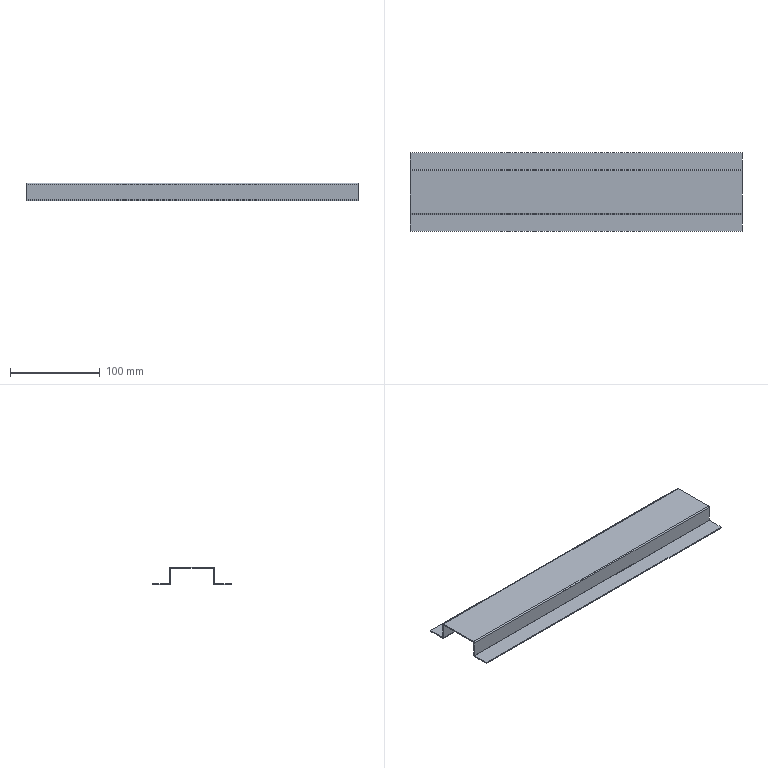Component | SolidWorks | WeldmentDrawing-1_FrontCrossbeam-1 | 1 solid | 38 faces | box 370 x 87.6 x 20 mm | volume 55055 mm3 | plane 30 | cylinder 8 | commonest cylinder face diameters 2.6 x4 0.2 x4
STEP:
#1=CARTESIAN_POINT('',(6.029,-6.77,9.791));
#2=VERTEX_POINT('',#1);
#3=CARTESIAN_POINT('',(6.029,-6.77,9.106));
#4=VERTEX_POINT('',#3);
#5=CARTESIAN_POINT('',(6.029,-6.77,9.795));
#6=DIRECTION('',(0.,-0.,-1.));
#7=VECTOR('',#6,39.37);
#8=LINE('',#5,#7);
#9=EDGE_CURVE('',#2,#4,#8,.T.);
#10=ORIENTED_EDGE('',*,*,#9,.T.);
#11=CARTESIAN_POINT('',(6.029,-6.723,9.106));
#12=VERTEX_POINT('',#11);
#13=CARTESIAN_POINT('',(6.029,-6.77,9.106));
#14=DIRECTION('',(0.,1.,0.));
#15=VECTOR('',#14,39.37);
#16=LINE('',#13,#15);
#17=EDGE_CURVE('',#4,#12,#16,.T.);
#18=ORIENTED_EDGE('',*,*,#17,.T.);
#19=CARTESIAN_POINT('',(6.029,-6.723,9.791));
#20=VERTEX_POINT('',#19);
#21=CARTESIAN_POINT('',(6.029,-6.723,9.843));
#22=DIRECTION('',(0.,-0.,-1.));
#23=VECTOR('',#22,39.37);
#24=LINE('',#21,#23);
#25=EDGE_CURVE('',#20,#12,#24,.T.);
#26=ORIENTED_EDGE('',*,*,#25,.F.);
#27=CARTESIAN_POINT('',(6.029,-6.77,9.791));
#28=DIRECTION('',(0.,-1.,0.));
#29=VECTOR('',#28,39.37);
#30=LINE('',#27,#29);
#31=EDGE_CURVE('',#20,#2,#30,.T.);
#32=ORIENTED_EDGE('',*,*,#31,.T.);
#33=EDGE_LOOP('',(#10,#18,#26,#32));
#34=FACE_OUTER_BOUND('',#33,.T.);
#35=CARTESIAN_POINT('',(6.029,-6.77,9.795));
#36=DIRECTION('',(1.,0.,0.));
#37=DIRECTION('',(0.,0.,-1.));
#38=AXIS2_PLACEMENT_3D('',#35,#36,#37);
#39=PLANE('',#38);
#40=ADVANCED_FACE('',(#34),#39,.T.);
#41=CARTESIAN_POINT('',(-8.538,-6.77,9.106));
#42=VERTEX_POINT('',#41);
#43=CARTESIAN_POINT('',(6.029,-6.77,9.106));
#44=DIRECTION('',(-1.,0.,0.));
#45=VECTOR('',#44,39.37);
#46=LINE('',#43,#45);
#47=EDGE_CURVE('',#4,#42,#46,.T.);
#48=ORIENTED_EDGE('',*,*,#47,.F.);
#49=ORIENTED_EDGE('',*,*,#9,.F.);
#50=CARTESIAN_POINT('',(-8.538,-6.77,9.791));
#51=VERTEX_POINT('',#50);
#52=CARTESIAN_POINT('',(6.029,-6.77,9.791));
#53=DIRECTION('',(1.,-0.,-0.));
#54=VECTOR('',#53,39.37);
#55=LINE('',#52,#54);
#56=EDGE_CURVE('',#51,#2,#55,.T.);
#57=ORIENTED_EDGE('',*,*,#56,.F.);
#58=CARTESIAN_POINT('',(-8.538,-6.77,9.055));
#59=DIRECTION('',(0.,0.,1.));
#60=VECTOR('',#59,39.37);
#61=LINE('',#58,#60);
#62=EDGE_CURVE('',#42,#51,#61,.T.);
#63=ORIENTED_EDGE('',*,*,#62,.F.);
#64=EDGE_LOOP('',(#48,#49,#57,#63));
#65=FACE_OUTER_BOUND('',#64,.T.);
#66=CARTESIAN_POINT('',(-5.572,-6.77,9.843));
#67=DIRECTION('',(0.,1.,-0.));
#68=DIRECTION('',(0.,0.,1.));
#69=AXIS2_PLACEMENT_3D('',#66,#67,#68);
#70=PLANE('',#69);
#71=ADVANCED_FACE('',(#65),#70,.F.);
#72=ORIENTED_EDGE('',*,*,#25,.T.);
#73=CARTESIAN_POINT('',(-8.538,-6.723,9.106));
#74=VERTEX_POINT('',#73);
#75=CARTESIAN_POINT('',(6.029,-6.723,9.106));
#76=DIRECTION('',(-1.,0.,0.));
#77=VECTOR('',#76,39.37);
#78=LINE('',#75,#77);
#79=EDGE_CURVE('',#12,#74,#78,.T.);
#80=ORIENTED_EDGE('',*,*,#79,.T.);
#81=CARTESIAN_POINT('',(-8.538,-6.723,9.791));
#82=VERTEX_POINT('',#81);
#83=CARTESIAN_POINT('',(-8.538,-6.723,9.843));
#84=DIRECTION('',(0.,0.,1.));
#85=VECTOR('',#84,39.37);
#86=LINE('',#83,#85);
#87=EDGE_CURVE('',#74,#82,#86,.T.);
#88=ORIENTED_EDGE('',*,*,#87,.T.);
#89=CARTESIAN_POINT('',(6.029,-6.723,9.791));
#90=DIRECTION('',(-1.,0.,0.));
#91=VECTOR('',#90,39.37);
#92=LINE('',#89,#91);
#93=EDGE_CURVE('',#20,#82,#92,.T.);
#94=ORIENTED_EDGE('',*,*,#93,.F.);
#95=EDGE_LOOP('',(#72,#80,#88,#94));
#96=FACE_OUTER_BOUND('',#95,.T.);
#97=CARTESIAN_POINT('',(-5.572,-6.723,9.843));
#98=DIRECTION('',(0.,1.,-0.));
#99=DIRECTION('',(0.,0.,1.));
#100=AXIS2_PLACEMENT_3D('',#97,#98,#99);
#101=PLANE('',#100);
#102=ADVANCED_FACE('',(#96),#101,.T.);
#103=CARTESIAN_POINT('',(-8.538,-4.801,9.791));
#104=VERTEX_POINT('',#103);
#105=CARTESIAN_POINT('',(-8.538,-4.801,9.106));
#106=VERTEX_POINT('',#105);
#107=CARTESIAN_POINT('',(-8.538,-4.801,9.055));
#108=DIRECTION('',(0.,0.,-1.));
#109=VECTOR('',#108,39.37);
#110=LINE('',#107,#109);
#111=EDGE_CURVE('',#104,#106,#110,.T.);
#112=ORIENTED_EDGE('',*,*,#111,.T.);
#113=CARTESIAN_POINT('',(-8.538,-4.848,9.106));
#114=VERTEX_POINT('',#113);
#115=CARTESIAN_POINT('',(-8.538,-4.801,9.106));
#116=DIRECTION('',(0.,-1.,0.));
#117=VECTOR('',#116,39.37);
#118=LINE('',#115,#117);
#119=EDGE_CURVE('',#106,#114,#118,.T.);
#120=ORIENTED_EDGE('',*,*,#119,.T.);
#121=CARTESIAN_POINT('',(-8.538,-4.848,9.791));
#122=VERTEX_POINT('',#121);
#123=CARTESIAN_POINT('',(-8.538,-4.848,9.843));
#124=DIRECTION('',(0.,0.,-1.));
#125=VECTOR('',#124,39.37);
#126=LINE('',#123,#125);
#127=EDGE_CURVE('',#122,#114,#126,.T.);
#128=ORIENTED_EDGE('',*,*,#127,.F.);
#129=CARTESIAN_POINT('',(-8.538,-4.801,9.791));
#130=DIRECTION('',(0.,1.,0.));
#131=VECTOR('',#130,39.37);
#132=LINE('',#129,#131);
#133=EDGE_CURVE('',#122,#104,#132,.T.);
#134=ORIENTED_EDGE('',*,*,#133,.T.);
#135=EDGE_LOOP('',(#112,#120,#128,#134));
#136=FACE_OUTER_BOUND('',#135,.T.);
#137=CARTESIAN_POINT('',(-8.538,-4.801,9.055));
#138=DIRECTION('',(-1.,0.,0.));
#139=DIRECTION('',(0.,0.,1.));
#140=AXIS2_PLACEMENT_3D('',#137,#138,#139);
#141=PLANE('',#140);
#142=ADVANCED_FACE('',(#136),#141,.T.);
#143=CARTESIAN_POINT('',(6.029,-4.801,9.106));
#144=VERTEX_POINT('',#143);
#145=CARTESIAN_POINT('',(6.029,-4.801,9.791));
#146=VERTEX_POINT('',#145);
#147=CARTESIAN_POINT('',(6.029,-4.801,9.795));
#148=DIRECTION('',(0.,-0.,1.));
#149=VECTOR('',#148,39.37);
#150=LINE('',#147,#149);
#151=EDGE_CURVE('',#144,#146,#150,.T.);
#152=ORIENTED_EDGE('',*,*,#151,.F.);
#153=CARTESIAN_POINT('',(-8.538,-4.801,9.106));
#154=DIRECTION('',(1.,0.,0.));
#155=VECTOR('',#154,39.37);
#156=LINE('',#153,#155);
#157=EDGE_CURVE('',#106,#144,#156,.T.);
#158=ORIENTED_EDGE('',*,*,#157,.F.);
#159=ORIENTED_EDGE('',*,*,#111,.F.);
#160=CARTESIAN_POINT('',(-5.572,-4.801,9.791));
#161=DIRECTION('',(1.,0.,-0.));
#162=VECTOR('',#161,39.37);
#163=LINE('',#160,#162);
#164=EDGE_CURVE('',#104,#146,#163,.T.);
#165=ORIENTED_EDGE('',*,*,#164,.T.);
#166=EDGE_LOOP('',(#152,#158,#159,#165));
#167=FACE_OUTER_BOUND('',#166,.T.);
#168=CARTESIAN_POINT('',(-5.572,-4.801,9.843));
#169=DIRECTION('',(0.,1.,0.));
#170=DIRECTION('',(0.,-0.,1.));
#171=AXIS2_PLACEMENT_3D('',#168,#169,#170);
#172=PLANE('',#171);
#173=ADVANCED_FACE('',(#167),#172,.T.);
#174=CARTESIAN_POINT('',(6.029,-4.848,9.106));
#175=VERTEX_POINT('',#174);
#176=CARTESIAN_POINT('',(-8.538,-4.848,9.106));
#177=DIRECTION('',(1.,0.,0.));
#178=VECTOR('',#177,39.37);
#179=LINE('',#176,#178);
#180=EDGE_CURVE('',#114,#175,#179,.T.);
#181=ORIENTED_EDGE('',*,*,#180,.T.);
#182=CARTESIAN_POINT('',(6.029,-4.848,9.791));
#183=VERTEX_POINT('',#182);
#184=CARTESIAN_POINT('',(6.029,-4.848,9.843));
#185=DIRECTION('',(0.,-0.,1.));
#186=VECTOR('',#185,39.37);
#187=LINE('',#184,#186);
#188=EDGE_CURVE('',#175,#183,#187,.T.);
#189=ORIENTED_EDGE('',*,*,#188,.T.);
#190=CARTESIAN_POINT('',(-8.538,-4.848,9.791));
#191=DIRECTION('',(1.,0.,-0.));
#192=VECTOR('',#191,39.37);
#193=LINE('',#190,#192);
#194=EDGE_CURVE('',#122,#183,#193,.T.);
#195=ORIENTED_EDGE('',*,*,#194,.F.);
#196=ORIENTED_EDGE('',*,*,#127,.T.);
#197=EDGE_LOOP('',(#181,#189,#195,#196));
#198=FACE_OUTER_BOUND('',#197,.T.);
#199=CARTESIAN_POINT('',(-5.572,-4.848,9.843));
#200=DIRECTION('',(0.,1.,0.));
#201=DIRECTION('',(0.,-0.,1.));
#202=AXIS2_PLACEMENT_3D('',#199,#200,#201);
#203=PLANE('',#202);
#204=ADVANCED_FACE('',(#198),#203,.F.);
#205=CARTESIAN_POINT('',(6.029,-6.719,9.795));
#206=VERTEX_POINT('',#205);
#207=CARTESIAN_POINT('',(6.029,-4.852,9.795));
#208=VERTEX_POINT('',#207);
#209=CARTESIAN_POINT('',(6.029,-6.77,9.795));
#210=DIRECTION('',(0.,1.,0.));
#211=VECTOR('',#210,39.37);
#212=LINE('',#209,#211);
#213=EDGE_CURVE('',#206,#208,#212,.T.);
#214=ORIENTED_EDGE('',*,*,#213,.F.);
#215=CARTESIAN_POINT('',(-8.538,-6.719,9.795));
#216=VERTEX_POINT('',#215);
#217=CARTESIAN_POINT('',(-8.538,-6.719,9.795));
#218=DIRECTION('',(1.,0.,0.));
#219=VECTOR('',#218,39.37);
#220=LINE('',#217,#219);
#221=EDGE_CURVE('',#216,#206,#220,.T.);
#222=ORIENTED_EDGE('',*,*,#221,.F.);
#223=CARTESIAN_POINT('',(-8.538,-4.852,9.795));
#224=VERTEX_POINT('',#223);
#225=CARTESIAN_POINT('',(-8.538,-6.77,9.795));
#226=DIRECTION('',(0.,-1.,0.));
#227=VECTOR('',#226,39.37);
#228=LINE('',#225,#227);
#229=EDGE_CURVE('',#224,#216,#228,.T.);
#230=ORIENTED_EDGE('',*,*,#229,.F.);
#231=CARTESIAN_POINT('',(6.029,-4.852,9.795));
#232=DIRECTION('',(-1.,0.,0.));
#233=VECTOR('',#232,39.37);
#234=LINE('',#231,#233);
#235=EDGE_CURVE('',#208,#224,#234,.T.);
#236=ORIENTED_EDGE('',*,*,#235,.F.);
#237=EDGE_LOOP('',(#214,#222,#230,#236));
#238=FACE_OUTER_BOUND('',#237,.T.);
#239=CARTESIAN_POINT('',(-5.572,-6.661,9.795));
#240=DIRECTION('',(0.,0.,-1.));
#241=DIRECTION('',(-1.,0.,0.));
#242=AXIS2_PLACEMENT_3D('',#239,#240,#241);
#243=PLANE('',#242);
#244=ADVANCED_FACE('',(#238),#243,.T.);
#245=CARTESIAN_POINT('',(-8.538,-6.719,9.843));
#246=VERTEX_POINT('',#245);
#247=CARTESIAN_POINT('',(6.029,-6.719,9.843));
#248=VERTEX_POINT('',#247);
#249=CARTESIAN_POINT('',(-8.538,-6.719,9.843));
#250=DIRECTION('',(1.,0.,0.));
#251=VECTOR('',#250,39.37);
#252=LINE('',#249,#251);
#253=EDGE_CURVE('',#246,#248,#252,.T.);
#254=ORIENTED_EDGE('',*,*,#253,.T.);
#255=CARTESIAN_POINT('',(6.029,-4.852,9.843));
#256=VERTEX_POINT('',#255);
#257=CARTESIAN_POINT('',(6.029,-6.77,9.843));
#258=DIRECTION('',(0.,1.,0.));
#259=VECTOR('',#258,39.37);
#260=LINE('',#257,#259);
#261=EDGE_CURVE('',#248,#256,#260,.T.);
#262=ORIENTED_EDGE('',*,*,#261,.T.);
#263=CARTESIAN_POINT('',(-8.538,-4.852,9.843));
#264=VERTEX_POINT('',#263);
#265=CARTESIAN_POINT('',(6.029,-4.852,9.843));
#266=DIRECTION('',(-1.,0.,0.));
#267=VECTOR('',#266,39.37);
#268=LINE('',#265,#267);
#269=EDGE_CURVE('',#256,#264,#268,.T.);
#270=ORIENTED_EDGE('',*,*,#269,.T.);
#271=CARTESIAN_POINT('',(-8.538,-6.77,9.843));
#272=DIRECTION('',(0.,-1.,0.));
#273=VECTOR('',#272,39.37);
#274=LINE('',#271,#273);
#275=EDGE_CURVE('',#264,#246,#274,.T.);
#276=ORIENTED_EDGE('',*,*,#275,.T.);
#277=EDGE_LOOP('',(#254,#262,#270,#276));
#278=FACE_OUTER_BOUND('',#277,.T.);
#279=CARTESIAN_POINT('',(-5.572,-6.661,9.843));
#280=DIRECTION('',(0.,0.,-1.));
#281=DIRECTION('',(-1.,0.,0.));
#282=AXIS2_PLACEMENT_3D('',#279,#280,#281);
#283=PLANE('',#282);
#284=ADVANCED_FACE('',(#278),#283,.F.);
#285=ORIENTED_EDGE('',*,*,#229,.T.);
#286=CARTESIAN_POINT('',(-8.538,-6.719,9.795));
#287=DIRECTION('',(0.,0.,1.));
#288=VECTOR('',#287,39.37);
#289=LINE('',#286,#288);
#290=EDGE_CURVE('',#216,#246,#289,.T.);
#291=ORIENTED_EDGE('',*,*,#290,.T.);
#292=ORIENTED_EDGE('',*,*,#275,.F.);
#293=CARTESIAN_POINT('',(-8.538,-4.852,9.795));
#294=DIRECTION('',(0.,0.,1.));
#295=VECTOR('',#294,39.37);
#296=LINE('',#293,#295);
#297=EDGE_CURVE('',#224,#264,#296,.T.);
#298=ORIENTED_EDGE('',*,*,#297,.F.);
#299=EDGE_LOOP('',(#285,#291,#292,#298));
#300=FACE_OUTER_BOUND('',#299,.T.);
#301=CARTESIAN_POINT('',(-8.538,-6.77,9.795));
#302=DIRECTION('',(-1.,0.,0.));
#303=DIRECTION('',(0.,0.,1.));
#304=AXIS2_PLACEMENT_3D('',#301,#302,#303);
#305=PLANE('',#304);
#306=ADVANCED_FACE('',(#300),#305,.T.);
#307=CARTESIAN_POINT('',(6.029,-6.719,9.795));
#308=DIRECTION('',(0.,0.,1.));
#309=VECTOR('',#308,39.37);
#310=LINE('',#307,#309);
#311=EDGE_CURVE('',#206,#248,#310,.T.);
#312=ORIENTED_EDGE('',*,*,#311,.F.);
#313=ORIENTED_EDGE('',*,*,#213,.T.);
#314=CARTESIAN_POINT('',(6.029,-4.852,9.795));
#315=DIRECTION('',(0.,0.,1.));
#316=VECTOR('',#315,39.37);
#317=LINE('',#314,#316);
#318=EDGE_CURVE('',#208,#256,#317,.T.);
#319=ORIENTED_EDGE('',*,*,#318,.T.);
#320=ORIENTED_EDGE('',*,*,#261,.F.);
#321=EDGE_LOOP('',(#312,#313,#319,#320));
#322=FACE_OUTER_BOUND('',#321,.T.);
#323=CARTESIAN_POINT('',(6.029,-6.77,9.795));
#324=DIRECTION('',(1.,0.,0.));
#325=DIRECTION('',(0.,0.,-1.));
#326=AXIS2_PLACEMENT_3D('',#323,#324,#325);
#327=PLANE('',#326);
#328=ADVANCED_FACE('',(#322),#327,.T.);
#329=ORIENTED_EDGE('',*,*,#133,.F.);
#330=CARTESIAN_POINT('',(-8.538,-4.852,9.791));
#331=DIRECTION('',(-1.,0.,0.));
#332=DIRECTION('',(0.,0.,-1.));
#333=AXIS2_PLACEMENT_3D('',#330,#331,#332);
#334=CIRCLE('',#333,0.003937);
#335=EDGE_CURVE('',#224,#122,#334,.T.);
#336=ORIENTED_EDGE('',*,*,#335,.F.);
#337=ORIENTED_EDGE('',*,*,#297,.T.);
#338=CARTESIAN_POINT('',(-8.538,-4.852,9.791));
#339=DIRECTION('',(-1.,0.,0.));
#340=DIRECTION('',(0.,0.,-1.));
#341=AXIS2_PLACEMENT_3D('',#338,#339,#340);
#342=CIRCLE('',#341,0.05118);
#343=EDGE_CURVE('',#264,#104,#342,.T.);
#344=ORIENTED_EDGE('',*,*,#343,.T.);
#345=EDGE_LOOP('',(#329,#336,#337,#344));
#346=FACE_OUTER_BOUND('',#345,.T.);
#347=CARTESIAN_POINT('',(-8.538,-4.852,9.791));
#348=DIRECTION('',(-1.,0.,0.));
#349=DIRECTION('',(0.,0.,1.));
#350=AXIS2_PLACEMENT_3D('',#347,#348,#349);
#351=PLANE('',#350);
#352=ADVANCED_FACE('',(#346),#351,.T.);
#353=CARTESIAN_POINT('',(6.029,-4.852,9.791));
#354=DIRECTION('',(1.,0.,0.));
#355=DIRECTION('',(0.,0.,-1.));
#356=AXIS2_PLACEMENT_3D('',#353,#354,#355);
#357=CIRCLE('',#356,0.003937);
#358=EDGE_CURVE('',#183,#208,#357,.T.);
#359=ORIENTED_EDGE('',*,*,#358,.F.);
#360=CARTESIAN_POINT('',(6.029,-4.848,9.791));
#361=DIRECTION('',(0.,1.,0.));
#362=VECTOR('',#361,39.37);
#363=LINE('',#360,#362);
#364=EDGE_CURVE('',#183,#146,#363,.T.);
#365=ORIENTED_EDGE('',*,*,#364,.T.);
#366=CARTESIAN_POINT('',(6.029,-4.852,9.791));
#367=DIRECTION('',(1.,0.,0.));
#368=DIRECTION('',(0.,0.,-1.));
#369=AXIS2_PLACEMENT_3D('',#366,#367,#368);
#370=CIRCLE('',#369,0.05118);
#371=EDGE_CURVE('',#146,#256,#370,.T.);
#372=ORIENTED_EDGE('',*,*,#371,.T.);
#373=ORIENTED_EDGE('',*,*,#318,.F.);
#374=EDGE_LOOP('',(#359,#365,#372,#373));
#375=FACE_OUTER_BOUND('',#374,.T.);
#376=CARTESIAN_POINT('',(6.029,-4.852,9.791));
#377=DIRECTION('',(-1.,0.,0.));
#378=DIRECTION('',(0.,0.,1.));
#379=AXIS2_PLACEMENT_3D('',#376,#377,#378);
#380=PLANE('',#379);
#381=ADVANCED_FACE('',(#375),#380,.F.);
#382=ORIENTED_EDGE('',*,*,#269,.F.);
#383=ORIENTED_EDGE('',*,*,#371,.F.);
#384=ORIENTED_EDGE('',*,*,#164,.F.);
#385=ORIENTED_EDGE('',*,*,#343,.F.);
#386=EDGE_LOOP('',(#382,#383,#384,#385));
#387=FACE_OUTER_BOUND('',#386,.T.);
#388=CARTESIAN_POINT('',(6.029,-4.852,9.791));
#389=DIRECTION('',(1.,0.,0.));
#390=DIRECTION('',(0.,1.,0.));
#391=AXIS2_PLACEMENT_3D('',#388,#389,#390);
#392=CYLINDRICAL_SURFACE('',#391,0.05118);
#393=ADVANCED_FACE('',(#387),#392,.T.);
#394=ORIENTED_EDGE('',*,*,#235,.T.);
#395=ORIENTED_EDGE('',*,*,#335,.T.);
#396=ORIENTED_EDGE('',*,*,#194,.T.);
#397=ORIENTED_EDGE('',*,*,#358,.T.);
#398=EDGE_LOOP('',(#394,#395,#396,#397));
#399=FACE_OUTER_BOUND('',#398,.T.);
#400=CARTESIAN_POINT('',(6.029,-4.852,9.791));
#401=DIRECTION('',(1.,0.,0.));
#402=DIRECTION('',(0.,1.,0.));
#403=AXIS2_PLACEMENT_3D('',#400,#401,#402);
#404=CYLINDRICAL_SURFACE('',#403,0.003937);
#405=ADVANCED_FACE('',(#399),#404,.F.);
#406=CARTESIAN_POINT('',(6.029,-4.801,9.106));
#407=DIRECTION('',(0.,-1.,0.));
#408=VECTOR('',#407,39.37);
#409=LINE('',#406,#408);
#410=EDGE_CURVE('',#144,#175,#409,.T.);
#411=ORIENTED_EDGE('',*,*,#410,.F.);
#412=ORIENTED_EDGE('',*,*,#151,.T.);
#413=ORIENTED_EDGE('',*,*,#364,.F.);
#414=ORIENTED_EDGE('',*,*,#188,.F.);
#415=EDGE_LOOP('',(#411,#412,#413,#414));
#416=FACE_OUTER_BOUND('',#415,.T.);
#417=CARTESIAN_POINT('',(6.029,-4.801,9.795));
#418=DIRECTION('',(1.,0.,0.));
#419=DIRECTION('',(0.,0.,-1.));
#420=AXIS2_PLACEMENT_3D('',#417,#418,#419);
#421=PLANE('',#420);
#422=ADVANCED_FACE('',(#416),#421,.T.);
#423=ORIENTED_EDGE('',*,*,#31,.F.);
#424=CARTESIAN_POINT('',(6.029,-6.719,9.791));
#425=DIRECTION('',(1.,0.,0.));
#426=DIRECTION('',(0.,0.,1.));
#427=AXIS2_PLACEMENT_3D('',#424,#425,#426);
#428=CIRCLE('',#427,0.003937);
#429=EDGE_CURVE('',#206,#20,#428,.T.);
#430=ORIENTED_EDGE('',*,*,#429,.F.);
#431=ORIENTED_EDGE('',*,*,#311,.T.);
#432=CARTESIAN_POINT('',(6.029,-6.719,9.791));
#433=DIRECTION('',(1.,0.,0.));
#434=DIRECTION('',(0.,0.,1.));
#435=AXIS2_PLACEMENT_3D('',#432,#433,#434);
#436=CIRCLE('',#435,0.05118);
#437=EDGE_CURVE('',#248,#2,#436,.T.);
#438=ORIENTED_EDGE('',*,*,#437,.T.);
#439=EDGE_LOOP('',(#423,#430,#431,#438));
#440=FACE_OUTER_BOUND('',#439,.T.);
#441=CARTESIAN_POINT('',(6.029,-6.719,9.791));
#442=DIRECTION('',(1.,0.,0.));
#443=DIRECTION('',(0.,0.,-1.));
#444=AXIS2_PLACEMENT_3D('',#441,#442,#443);
#445=PLANE('',#444);
#446=ADVANCED_FACE('',(#440),#445,.T.);
#447=CARTESIAN_POINT('',(-8.538,-6.719,9.791));
#448=DIRECTION('',(-1.,0.,0.));
#449=DIRECTION('',(0.,0.,1.));
#450=AXIS2_PLACEMENT_3D('',#447,#448,#449);
#451=CIRCLE('',#450,0.003937);
#452=EDGE_CURVE('',#82,#216,#451,.T.);
#453=ORIENTED_EDGE('',*,*,#452,.F.);
#454=CARTESIAN_POINT('',(-8.538,-6.723,9.791));
#455=DIRECTION('',(0.,-1.,0.));
#456=VECTOR('',#455,39.37);
#457=LINE('',#454,#456);
#458=EDGE_CURVE('',#82,#51,#457,.T.);
#459=ORIENTED_EDGE('',*,*,#458,.T.);
#460=CARTESIAN_POINT('',(-8.538,-6.719,9.791));
#461=DIRECTION('',(-1.,0.,0.));
#462=DIRECTION('',(0.,0.,1.));
#463=AXIS2_PLACEMENT_3D('',#460,#461,#462);
#464=CIRCLE('',#463,0.05118);
#465=EDGE_CURVE('',#51,#246,#464,.T.);
#466=ORIENTED_EDGE('',*,*,#465,.T.);
#467=ORIENTED_EDGE('',*,*,#290,.F.);
#468=EDGE_LOOP('',(#453,#459,#466,#467));
#469=FACE_OUTER_BOUND('',#468,.T.);
#470=CARTESIAN_POINT('',(-8.538,-6.719,9.791));
#471=DIRECTION('',(1.,0.,0.));
#472=DIRECTION('',(0.,0.,-1.));
#473=AXIS2_PLACEMENT_3D('',#470,#471,#472);
#474=PLANE('',#473);
#475=ADVANCED_FACE('',(#469),#474,.F.);
#476=ORIENTED_EDGE('',*,*,#253,.F.);
#477=ORIENTED_EDGE('',*,*,#465,.F.);
#478=ORIENTED_EDGE('',*,*,#56,.T.);
#479=ORIENTED_EDGE('',*,*,#437,.F.);
#480=EDGE_LOOP('',(#476,#477,#478,#479));
#481=FACE_OUTER_BOUND('',#480,.T.);
#482=CARTESIAN_POINT('',(-8.538,-6.719,9.791));
#483=DIRECTION('',(-1.,0.,0.));
#484=DIRECTION('',(0.,-1.,0.));
#485=AXIS2_PLACEMENT_3D('',#482,#483,#484);
#486=CYLINDRICAL_SURFACE('',#485,0.05118);
#487=ADVANCED_FACE('',(#481),#486,.T.);
#488=ORIENTED_EDGE('',*,*,#221,.T.);
#489=ORIENTED_EDGE('',*,*,#429,.T.);
#490=ORIENTED_EDGE('',*,*,#93,.T.);
#491=ORIENTED_EDGE('',*,*,#452,.T.);
#492=EDGE_LOOP('',(#488,#489,#490,#491));
#493=FACE_OUTER_BOUND('',#492,.T.);
#494=CARTESIAN_POINT('',(-8.538,-6.719,9.791));
#495=DIRECTION('',(-1.,0.,0.));
#496=DIRECTION('',(0.,-1.,0.));
#497=AXIS2_PLACEMENT_3D('',#494,#495,#496);
#498=CYLINDRICAL_SURFACE('',#497,0.003937);
#499=ADVANCED_FACE('',(#493),#498,.F.);
#500=CARTESIAN_POINT('',(-8.538,-6.77,9.106));
#501=DIRECTION('',(0.,1.,0.));
#502=VECTOR('',#501,39.37);
#503=LINE('',#500,#502);
#504=EDGE_CURVE('',#42,#74,#503,.T.);
#505=ORIENTED_EDGE('',*,*,#504,.F.);
#506=ORIENTED_EDGE('',*,*,#62,.T.);
#507=ORIENTED_EDGE('',*,*,#458,.F.);
#508=ORIENTED_EDGE('',*,*,#87,.F.);
#509=EDGE_LOOP('',(#505,#506,#507,#508));
#510=FACE_OUTER_BOUND('',#509,.T.);
#511=CARTESIAN_POINT('',(-8.538,-6.77,9.055));
#512=DIRECTION('',(-1.,0.,0.));
#513=DIRECTION('',(0.,0.,1.));
#514=AXIS2_PLACEMENT_3D('',#511,#512,#513);
#515=PLANE('',#514);
#516=ADVANCED_FACE('',(#510),#515,.T.);
#517=CARTESIAN_POINT('',(6.029,-4.797,9.102));
#518=VERTEX_POINT('',#517);
#519=CARTESIAN_POINT('',(6.029,-4.797,9.055));
#520=VERTEX_POINT('',#519);
#521=CARTESIAN_POINT('',(6.029,-4.797,9.055));
#522=DIRECTION('',(0.,0.,-1.));
#523=VECTOR('',#522,39.37);
#524=LINE('',#521,#523);
#525=EDGE_CURVE('',#518,#520,#524,.T.);
#526=ORIENTED_EDGE('',*,*,#525,.F.);
#527=CARTESIAN_POINT('',(6.029,-4.797,9.106));
#528=DIRECTION('',(1.,0.,0.));
#529=DIRECTION('',(0.,0.,1.));
#530=AXIS2_PLACEMENT_3D('',#527,#528,#529);
#531=CIRCLE('',#530,0.003937);
#532=EDGE_CURVE('',#144,#518,#531,.T.);
#533=ORIENTED_EDGE('',*,*,#532,.F.);
#534=ORIENTED_EDGE('',*,*,#410,.T.);
#535=CARTESIAN_POINT('',(6.029,-4.797,9.106));
#536=DIRECTION('',(1.,0.,0.));
#537=DIRECTION('',(0.,0.,1.));
#538=AXIS2_PLACEMENT_3D('',#535,#536,#537);
#539=CIRCLE('',#538,0.05118);
#540=EDGE_CURVE('',#175,#520,#539,.T.);
#541=ORIENTED_EDGE('',*,*,#540,.T.);
#542=EDGE_LOOP('',(#526,#533,#534,#541));
#543=FACE_OUTER_BOUND('',#542,.T.);
#544=CARTESIAN_POINT('',(6.029,-4.797,9.106));
#545=DIRECTION('',(1.,0.,0.));
#546=DIRECTION('',(0.,0.,-1.));
#547=AXIS2_PLACEMENT_3D('',#544,#545,#546);
#548=PLANE('',#547);
#549=ADVANCED_FACE('',(#543),#548,.T.);
#550=CARTESIAN_POINT('',(-8.538,-4.797,9.102));
#551=VERTEX_POINT('',#550);
#552=CARTESIAN_POINT('',(-8.538,-4.797,9.106));
#553=DIRECTION('',(-1.,0.,0.));
#554=DIRECTION('',(0.,0.,1.));
#555=AXIS2_PLACEMENT_3D('',#552,#553,#554);
#556=CIRCLE('',#555,0.003937);
#557=EDGE_CURVE('',#551,#106,#556,.T.);
#558=ORIENTED_EDGE('',*,*,#557,.F.);
#559=CARTESIAN_POINT('',(-8.538,-4.797,9.055));
#560=VERTEX_POINT('',#559);
#561=CARTESIAN_POINT('',(-8.538,-4.797,9.102));
#562=DIRECTION('',(0.,0.,-1.));
#563=VECTOR('',#562,39.37);
#564=LINE('',#561,#563);
#565=EDGE_CURVE('',#551,#560,#564,.T.);
#566=ORIENTED_EDGE('',*,*,#565,.T.);
#567=CARTESIAN_POINT('',(-8.538,-4.797,9.106));
#568=DIRECTION('',(-1.,0.,0.));
#569=DIRECTION('',(0.,0.,1.));
#570=AXIS2_PLACEMENT_3D('',#567,#568,#569);
#571=CIRCLE('',#570,0.05118);
#572=EDGE_CURVE('',#560,#114,#571,.T.);
#573=ORIENTED_EDGE('',*,*,#572,.T.);
#574=ORIENTED_EDGE('',*,*,#119,.F.);
#575=EDGE_LOOP('',(#558,#566,#573,#574));
#576=FACE_OUTER_BOUND('',#575,.T.);
#577=CARTESIAN_POINT('',(-8.538,-4.797,9.106));
#578=DIRECTION('',(1.,0.,0.));
#579=DIRECTION('',(0.,0.,-1.));
#580=AXIS2_PLACEMENT_3D('',#577,#578,#579);
#581=PLANE('',#580);
#582=ADVANCED_FACE('',(#576),#581,.F.);
#583=ORIENTED_EDGE('',*,*,#180,.F.);
#584=ORIENTED_EDGE('',*,*,#572,.F.);
#585=CARTESIAN_POINT('',(6.029,-4.797,9.055));
#586=DIRECTION('',(1.,0.,0.));
#587=VECTOR('',#586,39.37);
#588=LINE('',#585,#587);
#589=EDGE_CURVE('',#560,#520,#588,.T.);
#590=ORIENTED_EDGE('',*,*,#589,.T.);
#591=ORIENTED_EDGE('',*,*,#540,.F.);
#592=EDGE_LOOP('',(#583,#584,#590,#591));
#593=FACE_OUTER_BOUND('',#592,.T.);
#594=CARTESIAN_POINT('',(-8.538,-4.797,9.106));
#595=DIRECTION('',(-1.,0.,0.));
#596=DIRECTION('',(0.,0.,-1.));
#597=AXIS2_PLACEMENT_3D('',#594,#595,#596);
#598=CYLINDRICAL_SURFACE('',#597,0.05118);
#599=ADVANCED_FACE('',(#593),#598,.T.);
#600=ORIENTED_EDGE('',*,*,#157,.T.);
#601=ORIENTED_EDGE('',*,*,#532,.T.);
#602=CARTESIAN_POINT('',(6.029,-4.797,9.102));
#603=DIRECTION('',(-1.,0.,0.));
#604=VECTOR('',#603,39.37);
#605=LINE('',#602,#604);
#606=EDGE_CURVE('',#518,#551,#605,.T.);
#607=ORIENTED_EDGE('',*,*,#606,.T.);
#608=ORIENTED_EDGE('',*,*,#557,.T.);
#609=EDGE_LOOP('',(#600,#601,#607,#608));
#610=FACE_OUTER_BOUND('',#609,.T.);
#611=CARTESIAN_POINT('',(-8.538,-4.797,9.106));
#612=DIRECTION('',(-1.,0.,0.));
#613=DIRECTION('',(0.,0.,-1.));
#614=AXIS2_PLACEMENT_3D('',#611,#612,#613);
#615=CYLINDRICAL_SURFACE('',#614,0.003937);
#616=ADVANCED_FACE('',(#610),#615,.F.);
#617=ORIENTED_EDGE('',*,*,#565,.F.);
#618=CARTESIAN_POINT('',(-8.538,-4.061,9.102));
#619=VERTEX_POINT('',#618);
#620=CARTESIAN_POINT('',(-8.538,-4.061,9.102));
#621=DIRECTION('',(0.,1.,-0.));
#622=VECTOR('',#621,39.37);
#623=LINE('',#620,#622);
#624=EDGE_CURVE('',#551,#619,#623,.T.);
#625=ORIENTED_EDGE('',*,*,#624,.T.);
#626=CARTESIAN_POINT('',(-8.538,-4.061,9.055));
#627=VERTEX_POINT('',#626);
#628=CARTESIAN_POINT('',(-8.538,-4.061,9.055));
#629=DIRECTION('',(0.,0.,1.));
#630=VECTOR('',#629,39.37);
#631=LINE('',#628,#630);
#632=EDGE_CURVE('',#627,#619,#631,.T.);
#633=ORIENTED_EDGE('',*,*,#632,.F.);
#634=CARTESIAN_POINT('',(-8.538,-6.661,9.055));
#635=DIRECTION('',(0.,1.,-0.));
#636=VECTOR('',#635,39.37);
#637=LINE('',#634,#636);
#638=EDGE_CURVE('',#560,#627,#637,.T.);
#639=ORIENTED_EDGE('',*,*,#638,.F.);
#640=EDGE_LOOP('',(#617,#625,#633,#639));
#641=FACE_OUTER_BOUND('',#640,.T.);
#642=CARTESIAN_POINT('',(-8.538,-4.061,9.055));
#643=DIRECTION('',(1.,0.,0.));
#644=DIRECTION('',(0.,0.,-1.));
#645=AXIS2_PLACEMENT_3D('',#642,#643,#644);
#646=PLANE('',#645);
#647=ADVANCED_FACE('',(#641),#646,.F.);
#648=ORIENTED_EDGE('',*,*,#525,.T.);
#649=CARTESIAN_POINT('',(6.029,-4.061,9.055));
#650=VERTEX_POINT('',#649);
#651=CARTESIAN_POINT('',(6.029,-6.661,9.055));
#652=DIRECTION('',(0.,-1.,0.));
#653=VECTOR('',#652,39.37);
#654=LINE('',#651,#653);
#655=EDGE_CURVE('',#650,#520,#654,.T.);
#656=ORIENTED_EDGE('',*,*,#655,.F.);
#657=CARTESIAN_POINT('',(6.029,-4.061,9.102));
#658=VERTEX_POINT('',#657);
#659=CARTESIAN_POINT('',(6.029,-4.061,9.055));
#660=DIRECTION('',(0.,0.,1.));
#661=VECTOR('',#660,39.37);
#662=LINE('',#659,#661);
#663=EDGE_CURVE('',#650,#658,#662,.T.);
#664=ORIENTED_EDGE('',*,*,#663,.T.);
#665=CARTESIAN_POINT('',(6.029,-4.801,9.102));
#666=DIRECTION('',(0.,-1.,0.));
#667=VECTOR('',#666,39.37);
#668=LINE('',#665,#667);
#669=EDGE_CURVE('',#658,#518,#668,.T.);
#670=ORIENTED_EDGE('',*,*,#669,.T.);
#671=EDGE_LOOP('',(#648,#656,#664,#670));
#672=FACE_OUTER_BOUND('',#671,.T.);
#673=CARTESIAN_POINT('',(6.029,-4.801,9.055));
#674=DIRECTION('',(-1.,0.,0.));
#675=DIRECTION('',(0.,0.,1.));
#676=AXIS2_PLACEMENT_3D('',#673,#674,#675);
#677=PLANE('',#676);
#678=ADVANCED_FACE('',(#672),#677,.F.);
#679=ORIENTED_EDGE('',*,*,#589,.F.);
#680=ORIENTED_EDGE('',*,*,#638,.T.);
#681=CARTESIAN_POINT('',(-5.572,-4.061,9.055));
#682=DIRECTION('',(1.,0.,0.));
#683=VECTOR('',#682,39.37);
#684=LINE('',#681,#683);
#685=EDGE_CURVE('',#627,#650,#684,.T.);
#686=ORIENTED_EDGE('',*,*,#685,.T.);
#687=ORIENTED_EDGE('',*,*,#655,.T.);
#688=EDGE_LOOP('',(#679,#680,#686,#687));
#689=FACE_OUTER_BOUND('',#688,.T.);
#690=CARTESIAN_POINT('',(-5.572,-6.661,9.055));
#691=DIRECTION('',(0.,0.,1.));
#692=DIRECTION('',(0.,-1.,0.));
#693=AXIS2_PLACEMENT_3D('',#690,#691,#692);
#694=PLANE('',#693);
#695=ADVANCED_FACE('',(#689),#694,.F.);
#696=ORIENTED_EDGE('',*,*,#624,.F.);
#697=ORIENTED_EDGE('',*,*,#606,.F.);
#698=ORIENTED_EDGE('',*,*,#669,.F.);
#699=CARTESIAN_POINT('',(6.029,-4.061,9.102));
#700=DIRECTION('',(1.,0.,0.));
#701=VECTOR('',#700,39.37);
#702=LINE('',#699,#701);
#703=EDGE_CURVE('',#619,#658,#702,.T.);
#704=ORIENTED_EDGE('',*,*,#703,.F.);
#705=EDGE_LOOP('',(#696,#697,#698,#704));
#706=FACE_OUTER_BOUND('',#705,.T.);
#707=CARTESIAN_POINT('',(-5.572,-6.661,9.102));
#708=DIRECTION('',(0.,0.,1.));
#709=DIRECTION('',(0.,-1.,0.));
#710=AXIS2_PLACEMENT_3D('',#707,#708,#709);
#711=PLANE('',#710);
#712=ADVANCED_FACE('',(#706),#711,.T.);
#713=ORIENTED_EDGE('',*,*,#703,.T.);
#714=ORIENTED_EDGE('',*,*,#663,.F.);
#715=ORIENTED_EDGE('',*,*,#685,.F.);
#716=ORIENTED_EDGE('',*,*,#632,.T.);
#717=EDGE_LOOP('',(#713,#714,#715,#716));
#718=FACE_OUTER_BOUND('',#717,.T.);
#719=CARTESIAN_POINT('',(6.029,-4.061,9.055));
#720=DIRECTION('',(0.,-1.,0.));
#721=DIRECTION('',(0.,-0.,-1.));
#722=AXIS2_PLACEMENT_3D('',#719,#720,#721);
#723=PLANE('',#722);
#724=ADVANCED_FACE('',(#718),#723,.F.);
#725=CARTESIAN_POINT('',(-8.538,-6.774,9.102));
#726=VERTEX_POINT('',#725);
#727=CARTESIAN_POINT('',(-8.538,-6.774,9.055));
#728=VERTEX_POINT('',#727);
#729=CARTESIAN_POINT('',(-8.538,-6.774,9.055));
#730=DIRECTION('',(0.,0.,-1.));
#731=VECTOR('',#730,39.37);
#732=LINE('',#729,#731);
#733=EDGE_CURVE('',#726,#728,#732,.T.);
#734=ORIENTED_EDGE('',*,*,#733,.F.);
#735=CARTESIAN_POINT('',(-8.538,-6.774,9.106));
#736=DIRECTION('',(-1.,0.,0.));
#737=DIRECTION('',(0.,0.,-1.));
#738=AXIS2_PLACEMENT_3D('',#735,#736,#737);
#739=CIRCLE('',#738,0.003937);
#740=EDGE_CURVE('',#42,#726,#739,.T.);
#741=ORIENTED_EDGE('',*,*,#740,.F.);
#742=ORIENTED_EDGE('',*,*,#504,.T.);
#743=CARTESIAN_POINT('',(-8.538,-6.774,9.106));
#744=DIRECTION('',(-1.,0.,0.));
#745=DIRECTION('',(0.,0.,-1.));
#746=AXIS2_PLACEMENT_3D('',#743,#744,#745);
#747=CIRCLE('',#746,0.05118);
#748=EDGE_CURVE('',#74,#728,#747,.T.);
#749=ORIENTED_EDGE('',*,*,#748,.T.);
#750=EDGE_LOOP('',(#734,#741,#742,#749));
#751=FACE_OUTER_BOUND('',#750,.T.);
#752=CARTESIAN_POINT('',(-8.538,-6.774,9.106));
#753=DIRECTION('',(-1.,0.,0.));
#754=DIRECTION('',(0.,0.,1.));
#755=AXIS2_PLACEMENT_3D('',#752,#753,#754);
#756=PLANE('',#755);
#757=ADVANCED_FACE('',(#751),#756,.T.);
#758=CARTESIAN_POINT('',(6.029,-6.774,9.102));
#759=VERTEX_POINT('',#758);
#760=CARTESIAN_POINT('',(6.029,-6.774,9.106));
#761=DIRECTION('',(1.,0.,0.));
#762=DIRECTION('',(0.,0.,-1.));
#763=AXIS2_PLACEMENT_3D('',#760,#761,#762);
#764=CIRCLE('',#763,0.003937);
#765=EDGE_CURVE('',#759,#4,#764,.T.);
#766=ORIENTED_EDGE('',*,*,#765,.F.);
#767=CARTESIAN_POINT('',(6.029,-6.774,9.055));
#768=VERTEX_POINT('',#767);
#769=CARTESIAN_POINT('',(6.029,-6.774,9.102));
#770=DIRECTION('',(0.,0.,-1.));
#771=VECTOR('',#770,39.37);
#772=LINE('',#769,#771);
#773=EDGE_CURVE('',#759,#768,#772,.T.);
#774=ORIENTED_EDGE('',*,*,#773,.T.);
#775=CARTESIAN_POINT('',(6.029,-6.774,9.106));
#776=DIRECTION('',(1.,0.,0.));
#777=DIRECTION('',(0.,0.,-1.));
#778=AXIS2_PLACEMENT_3D('',#775,#776,#777);
#779=CIRCLE('',#778,0.05118);
#780=EDGE_CURVE('',#768,#12,#779,.T.);
#781=ORIENTED_EDGE('',*,*,#780,.T.);
#782=ORIENTED_EDGE('',*,*,#17,.F.);
#783=EDGE_LOOP('',(#766,#774,#781,#782));
#784=FACE_OUTER_BOUND('',#783,.T.);
#785=CARTESIAN_POINT('',(6.029,-6.774,9.106));
#786=DIRECTION('',(-1.,0.,0.));
#787=DIRECTION('',(0.,0.,1.));
#788=AXIS2_PLACEMENT_3D('',#785,#786,#787);
#789=PLANE('',#788);
#790=ADVANCED_FACE('',(#784),#789,.F.);
#791=ORIENTED_EDGE('',*,*,#79,.F.);
#792=ORIENTED_EDGE('',*,*,#780,.F.);
#793=CARTESIAN_POINT('',(-8.538,-6.774,9.055));
#794=DIRECTION('',(-1.,-0.,0.));
#795=VECTOR('',#794,39.37);
#796=LINE('',#793,#795);
#797=EDGE_CURVE('',#768,#728,#796,.T.);
#798=ORIENTED_EDGE('',*,*,#797,.T.);
#799=ORIENTED_EDGE('',*,*,#748,.F.);
#800=EDGE_LOOP('',(#791,#792,#798,#799));
#801=FACE_OUTER_BOUND('',#800,.T.);
#802=CARTESIAN_POINT('',(6.029,-6.774,9.106));
#803=DIRECTION('',(1.,0.,0.));
#804=DIRECTION('',(0.,0.,-1.));
#805=AXIS2_PLACEMENT_3D('',#802,#803,#804);
#806=CYLINDRICAL_SURFACE('',#805,0.05118);
#807=ADVANCED_FACE('',(#801),#806,.T.);
#808=ORIENTED_EDGE('',*,*,#47,.T.);
#809=ORIENTED_EDGE('',*,*,#740,.T.);
#810=CARTESIAN_POINT('',(-8.538,-6.774,9.102));
#811=DIRECTION('',(1.,0.,0.));
#812=VECTOR('',#811,39.37);
#813=LINE('',#810,#812);
#814=EDGE_CURVE('',#726,#759,#813,.T.);
#815=ORIENTED_EDGE('',*,*,#814,.T.);
#816=ORIENTED_EDGE('',*,*,#765,.T.);
#817=EDGE_LOOP('',(#808,#809,#815,#816));
#818=FACE_OUTER_BOUND('',#817,.T.);
#819=CARTESIAN_POINT('',(6.029,-6.774,9.106));
#820=DIRECTION('',(1.,0.,0.));
#821=DIRECTION('',(0.,0.,-1.));
#822=AXIS2_PLACEMENT_3D('',#819,#820,#821);
#823=CYLINDRICAL_SURFACE('',#822,0.003937);
#824=ADVANCED_FACE('',(#818),#823,.F.);
#825=ORIENTED_EDGE('',*,*,#773,.F.);
#826=CARTESIAN_POINT('',(6.029,-7.51,9.102));
#827=VERTEX_POINT('',#826);
#828=CARTESIAN_POINT('',(6.029,-7.51,9.102));
#829=DIRECTION('',(0.,-1.,0.));
#830=VECTOR('',#829,39.37);
#831=LINE('',#828,#830);
#832=EDGE_CURVE('',#759,#827,#831,.T.);
#833=ORIENTED_EDGE('',*,*,#832,.T.);
#834=CARTESIAN_POINT('',(6.029,-7.51,9.055));
#835=VERTEX_POINT('',#834);
#836=CARTESIAN_POINT('',(6.029,-7.51,9.055));
#837=DIRECTION('',(0.,-0.,1.));
#838=VECTOR('',#837,39.37);
#839=LINE('',#836,#838);
#840=EDGE_CURVE('',#835,#827,#839,.T.);
#841=ORIENTED_EDGE('',*,*,#840,.F.);
#842=CARTESIAN_POINT('',(6.029,-6.661,9.055));
#843=DIRECTION('',(0.,-1.,0.));
#844=VECTOR('',#843,39.37);
#845=LINE('',#842,#844);
#846=EDGE_CURVE('',#768,#835,#845,.T.);
#847=ORIENTED_EDGE('',*,*,#846,.F.);
#848=EDGE_LOOP('',(#825,#833,#841,#847));
#849=FACE_OUTER_BOUND('',#848,.T.);
#850=CARTESIAN_POINT('',(6.029,-7.51,9.055));
#851=DIRECTION('',(-1.,0.,0.));
#852=DIRECTION('',(0.,0.,1.));
#853=AXIS2_PLACEMENT_3D('',#850,#851,#852);
#854=PLANE('',#853);
#855=ADVANCED_FACE('',(#849),#854,.F.);
#856=ORIENTED_EDGE('',*,*,#733,.T.);
#857=CARTESIAN_POINT('',(-8.538,-7.51,9.055));
#858=VERTEX_POINT('',#857);
#859=CARTESIAN_POINT('',(-8.538,-6.661,9.055));
#860=DIRECTION('',(0.,1.,0.));
#861=VECTOR('',#860,39.37);
#862=LINE('',#859,#861);
#863=EDGE_CURVE('',#858,#728,#862,.T.);
#864=ORIENTED_EDGE('',*,*,#863,.F.);
#865=CARTESIAN_POINT('',(-8.538,-7.51,9.102));
#866=VERTEX_POINT('',#865);
#867=CARTESIAN_POINT('',(-8.538,-7.51,9.055));
#868=DIRECTION('',(0.,-0.,1.));
#869=VECTOR('',#868,39.37);
#870=LINE('',#867,#869);
#871=EDGE_CURVE('',#858,#866,#870,.T.);
#872=ORIENTED_EDGE('',*,*,#871,.T.);
#873=CARTESIAN_POINT('',(-8.538,-6.77,9.102));
#874=DIRECTION('',(0.,1.,0.));
#875=VECTOR('',#874,39.37);
#876=LINE('',#873,#875);
#877=EDGE_CURVE('',#866,#726,#876,.T.);
#878=ORIENTED_EDGE('',*,*,#877,.T.);
#879=EDGE_LOOP('',(#856,#864,#872,#878));
#880=FACE_OUTER_BOUND('',#879,.T.);
#881=CARTESIAN_POINT('',(-8.538,-6.77,9.055));
#882=DIRECTION('',(1.,0.,0.));
#883=DIRECTION('',(0.,0.,-1.));
#884=AXIS2_PLACEMENT_3D('',#881,#882,#883);
#885=PLANE('',#884);
#886=ADVANCED_FACE('',(#880),#885,.F.);
#887=ORIENTED_EDGE('',*,*,#797,.F.);
#888=ORIENTED_EDGE('',*,*,#846,.T.);
#889=CARTESIAN_POINT('',(-5.572,-7.51,9.055));
#890=DIRECTION('',(-1.,0.,0.));
#891=VECTOR('',#890,39.37);
#892=LINE('',#889,#891);
#893=EDGE_CURVE('',#835,#858,#892,.T.);
#894=ORIENTED_EDGE('',*,*,#893,.T.);
#895=ORIENTED_EDGE('',*,*,#863,.T.);
#896=EDGE_LOOP('',(#887,#888,#894,#895));
#897=FACE_OUTER_BOUND('',#896,.T.);
#898=CARTESIAN_POINT('',(-5.572,-6.661,9.055));
#899=DIRECTION('',(0.,0.,1.));
#900=DIRECTION('',(1.,0.,0.));
#901=AXIS2_PLACEMENT_3D('',#898,#899,#900);
#902=PLANE('',#901);
#903=ADVANCED_FACE('',(#897),#902,.F.);
#904=ORIENTED_EDGE('',*,*,#832,.F.);
#905=ORIENTED_EDGE('',*,*,#814,.F.);
#906=ORIENTED_EDGE('',*,*,#877,.F.);
#907=CARTESIAN_POINT('',(-8.538,-7.51,9.102));
#908=DIRECTION('',(-1.,0.,0.));
#909=VECTOR('',#908,39.37);
#910=LINE('',#907,#909);
#911=EDGE_CURVE('',#827,#866,#910,.T.);
#912=ORIENTED_EDGE('',*,*,#911,.F.);
#913=EDGE_LOOP('',(#904,#905,#906,#912));
#914=FACE_OUTER_BOUND('',#913,.T.);
#915=CARTESIAN_POINT('',(-5.572,-6.661,9.102));
#916=DIRECTION('',(0.,0.,1.));
#917=DIRECTION('',(1.,0.,0.));
#918=AXIS2_PLACEMENT_3D('',#915,#916,#917);
#919=PLANE('',#918);
#920=ADVANCED_FACE('',(#914),#919,.T.);
#921=ORIENTED_EDGE('',*,*,#911,.T.);
#922=ORIENTED_EDGE('',*,*,#871,.F.);
#923=ORIENTED_EDGE('',*,*,#893,.F.);
#924=ORIENTED_EDGE('',*,*,#840,.T.);
#925=EDGE_LOOP('',(#921,#922,#923,#924));
#926=FACE_OUTER_BOUND('',#925,.T.);
#927=CARTESIAN_POINT('',(-8.538,-7.51,9.055));
#928=DIRECTION('',(0.,1.,0.));
#929=DIRECTION('',(0.,-0.,1.));
#930=AXIS2_PLACEMENT_3D('',#927,#928,#929);
#931=PLANE('',#930);
#932=ADVANCED_FACE('',(#926),#931,.F.);
#933=CLOSED_SHELL('',(#40,#71,#102,#142,#173,#204,#244,#284,#306,#328,#352,#381,#393,#405,#422,#446,#475,#487,#499,#516,#549,#582,#599,#616,#647,#678,#695,#712,#724,#757,#790,#807,#824,#855,#886,#903,#920,#932));
#934=MANIFOLD_SOLID_BREP('',#933);
#935=CARTESIAN_POINT('',(0.,0.,0.));
#936=DIRECTION('',(0.,0.,1.));
#937=DIRECTION('',(1.,0.,0.));
#938=AXIS2_PLACEMENT_3D('',#935,#936,#937);
#939=(LENGTH_UNIT()NAMED_UNIT(*)SI_UNIT($,.METRE.));
#940=LENGTH_MEASURE_WITH_UNIT(LENGTH_MEASURE(0.0254),#939);
#941=DIMENSIONAL_EXPONENTS(1.,0.,0.,0.,0.,0.,0.);
#942=(CONVERSION_BASED_UNIT('',#940)LENGTH_UNIT()NAMED_UNIT(#941));
#943=UNCERTAINTY_MEASURE_WITH_UNIT(LENGTH_MEASURE(0.00001),#942,'','');
#944=(NAMED_UNIT(*)PLANE_ANGLE_UNIT()SI_UNIT($,.RADIAN.));
#945=(NAMED_UNIT(*)SI_UNIT($,.STERADIAN.)SOLID_ANGLE_UNIT());
#946=(GEOMETRIC_REPRESENTATION_CONTEXT(3)GLOBAL_UNCERTAINTY_ASSIGNED_CONTEXT((#943))GLOBAL_UNIT_ASSIGNED_CONTEXT((#942,#944,#945))REPRESENTATION_CONTEXT('',''));
#947=ADVANCED_BREP_SHAPE_REPRESENTATION('',(#934,#938),#946);
#948=COLOUR_RGB('',0.7922,0.8196,0.9333);
#949=FILL_AREA_STYLE_COLOUR('',#948);
#950=FILL_AREA_STYLE('',(#949));
#951=SURFACE_STYLE_FILL_AREA(#950);
#952=SURFACE_SIDE_STYLE('',(#951));
#953=SURFACE_STYLE_USAGE(.BOTH.,#952);
#954=PRESENTATION_STYLE_ASSIGNMENT((#953));
#955=STYLED_ITEM('',(#954),#934);
#956=PRESENTATION_LAYER_ASSIGNMENT('','',(#955));
#957=(LENGTH_UNIT()NAMED_UNIT(*)SI_UNIT($,.METRE.));
#958=LENGTH_MEASURE_WITH_UNIT(LENGTH_MEASURE(0.0254),#957);
#959=DIMENSIONAL_EXPONENTS(1.,0.,0.,0.,0.,0.,0.);
#960=(CONVERSION_BASED_UNIT('',#958)LENGTH_UNIT()NAMED_UNIT(#959));
#961=UNCERTAINTY_MEASURE_WITH_UNIT(LENGTH_MEASURE(0.00001),#960,'','');
#962=(NAMED_UNIT(*)PLANE_ANGLE_UNIT()SI_UNIT($,.RADIAN.));
#963=(NAMED_UNIT(*)SI_UNIT($,.STERADIAN.)SOLID_ANGLE_UNIT());
#964=(GEOMETRIC_REPRESENTATION_CONTEXT(3)GLOBAL_UNCERTAINTY_ASSIGNED_CONTEXT((#961))GLOBAL_UNIT_ASSIGNED_CONTEXT((#960,#962,#963))REPRESENTATION_CONTEXT('',''));
#965=MECHANICAL_DESIGN_GEOMETRIC_PRESENTATION_REPRESENTATION('',(#955),#964);